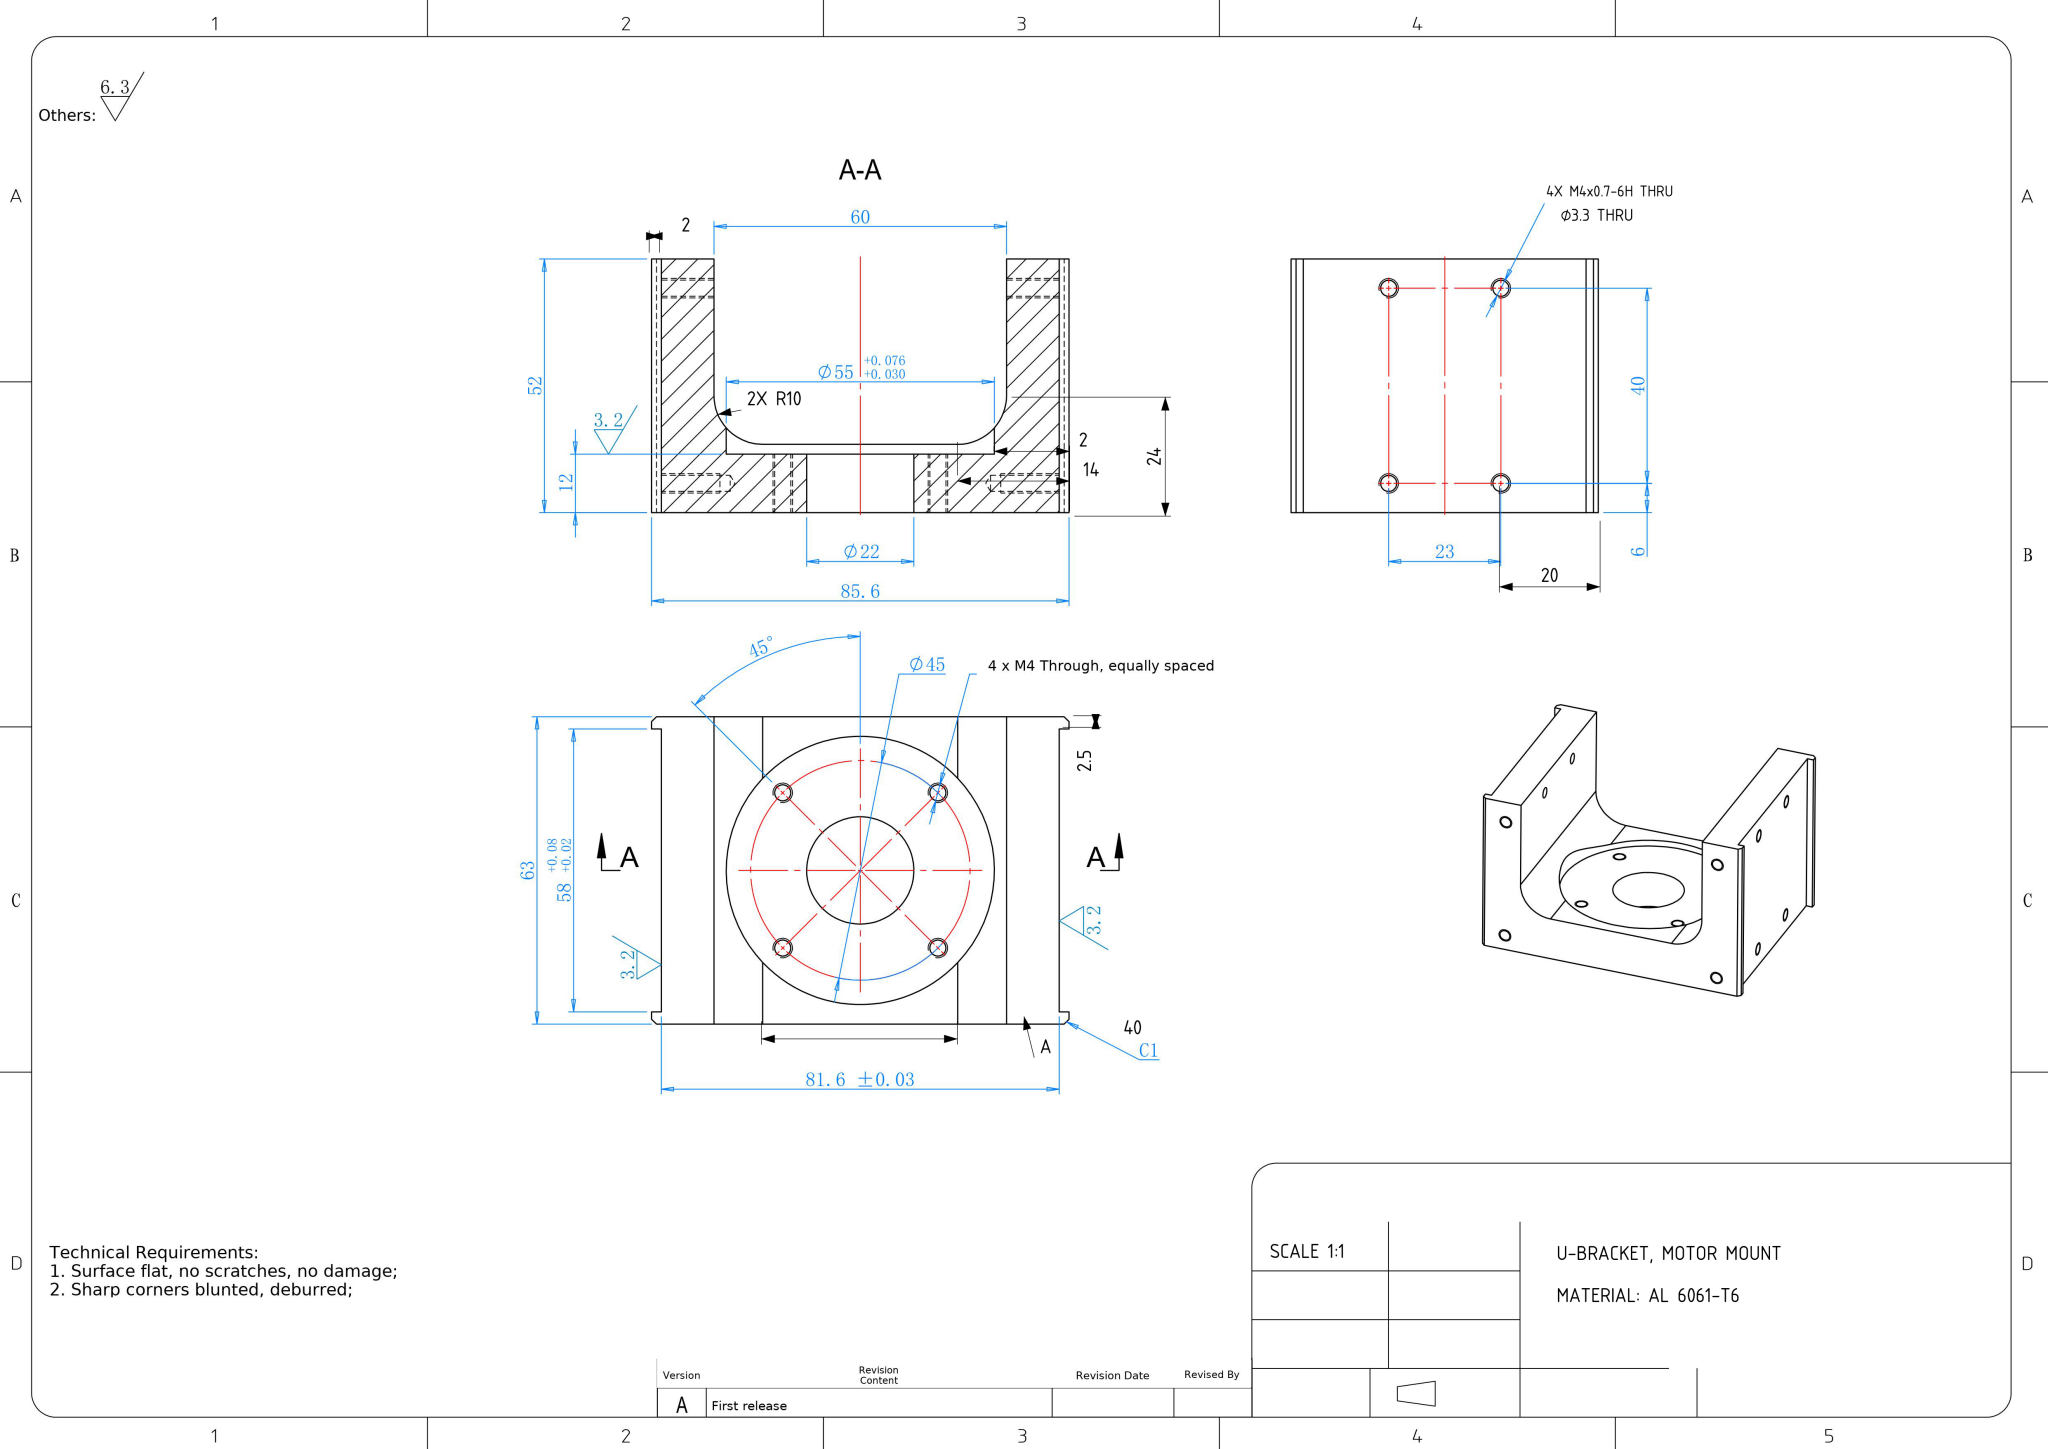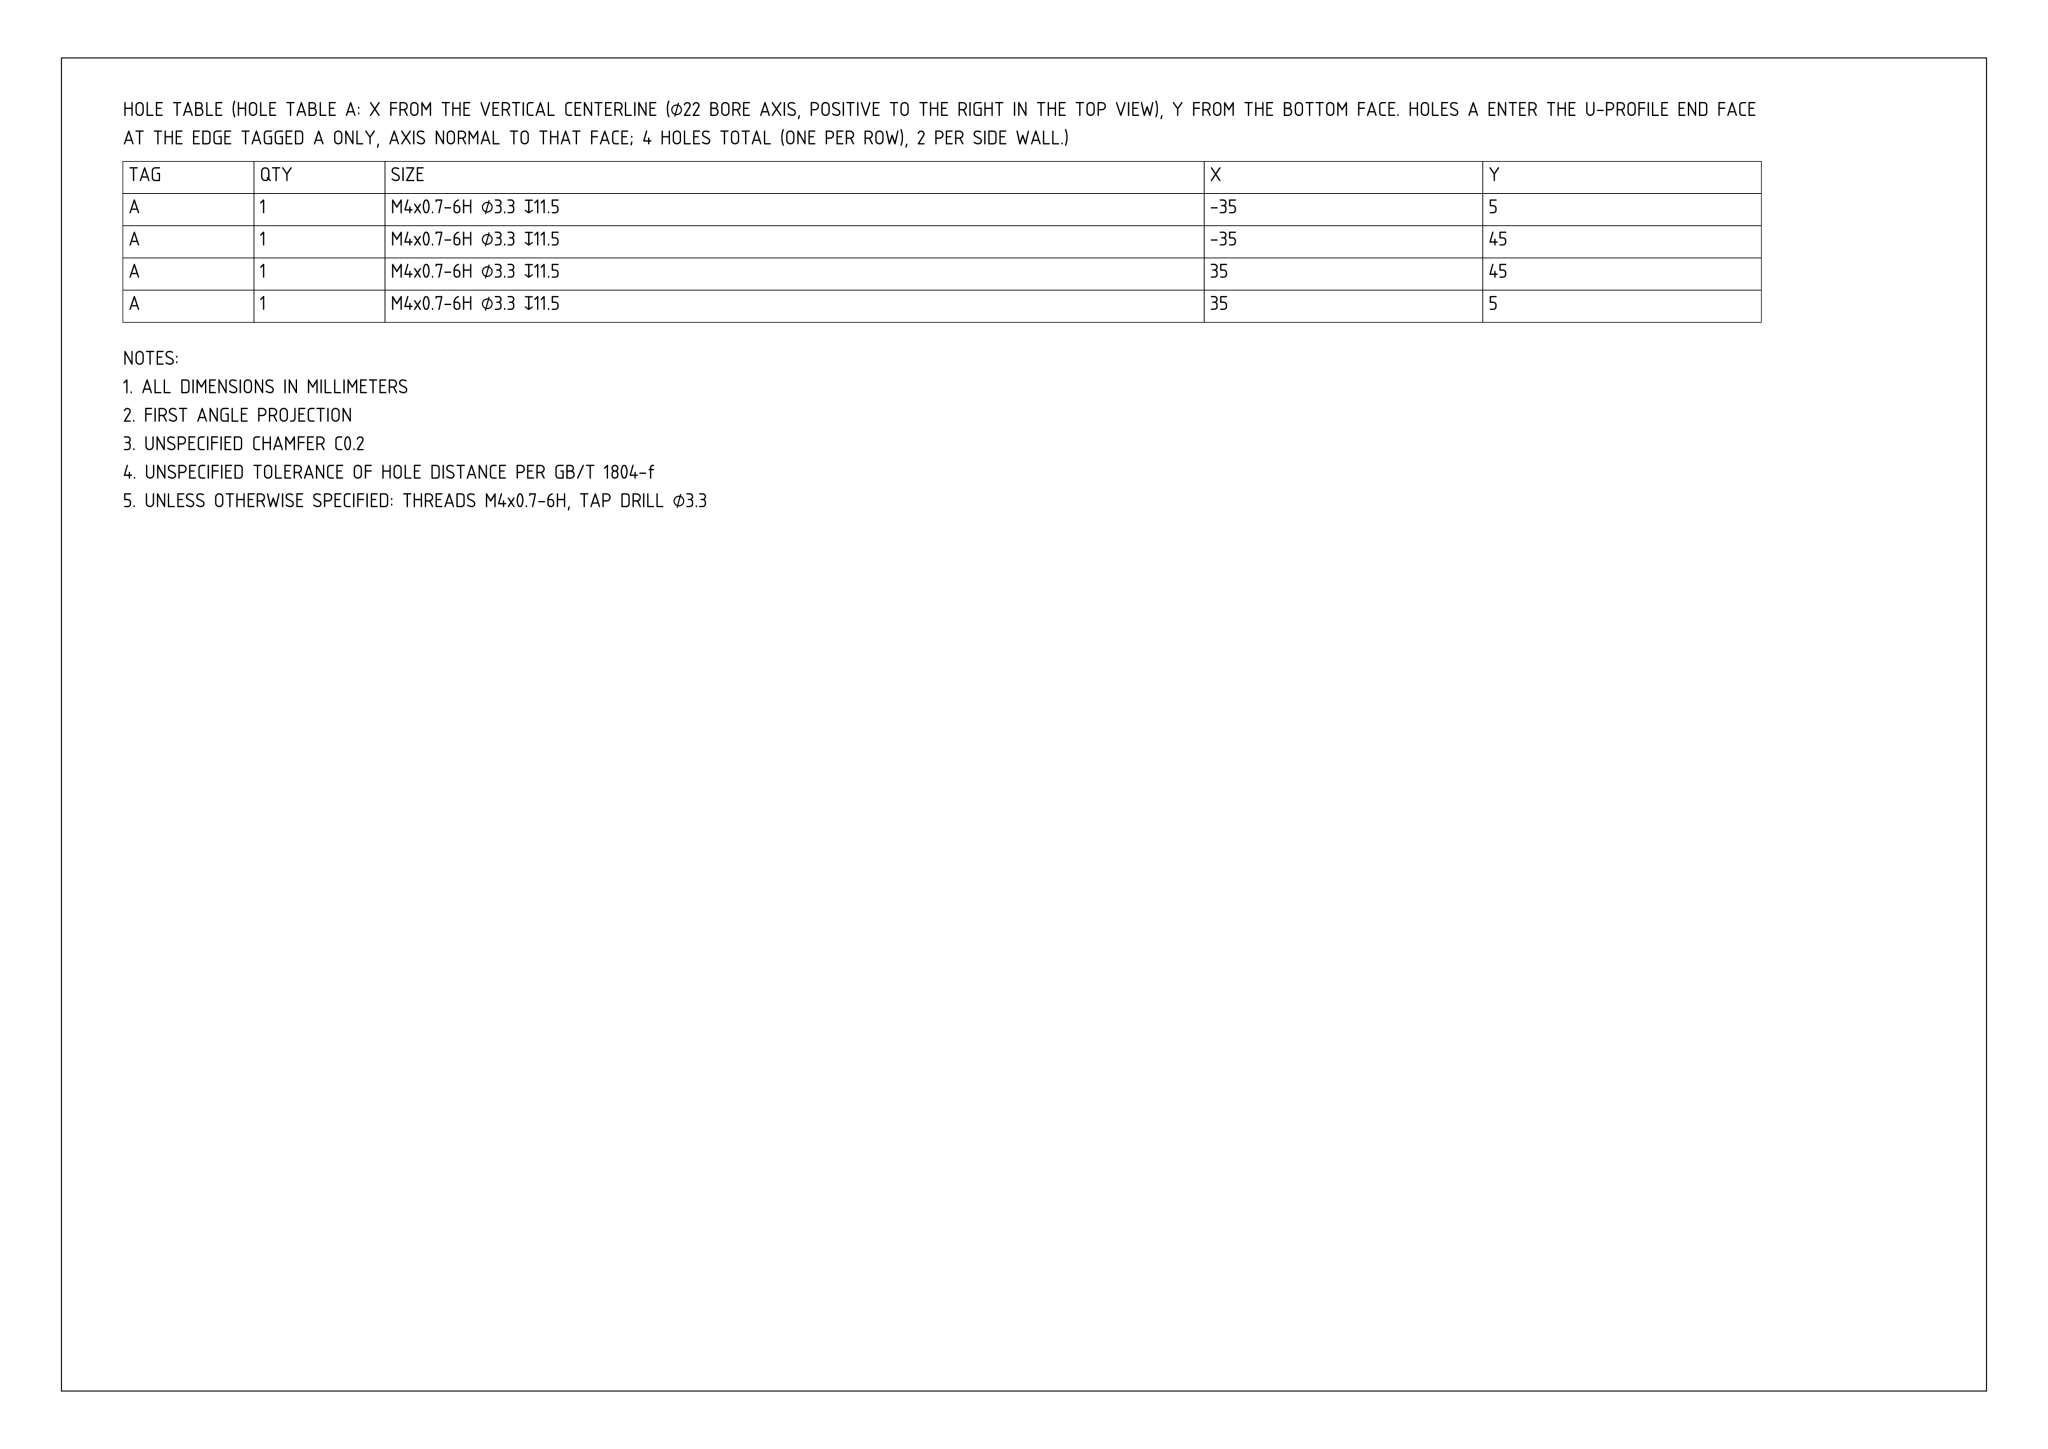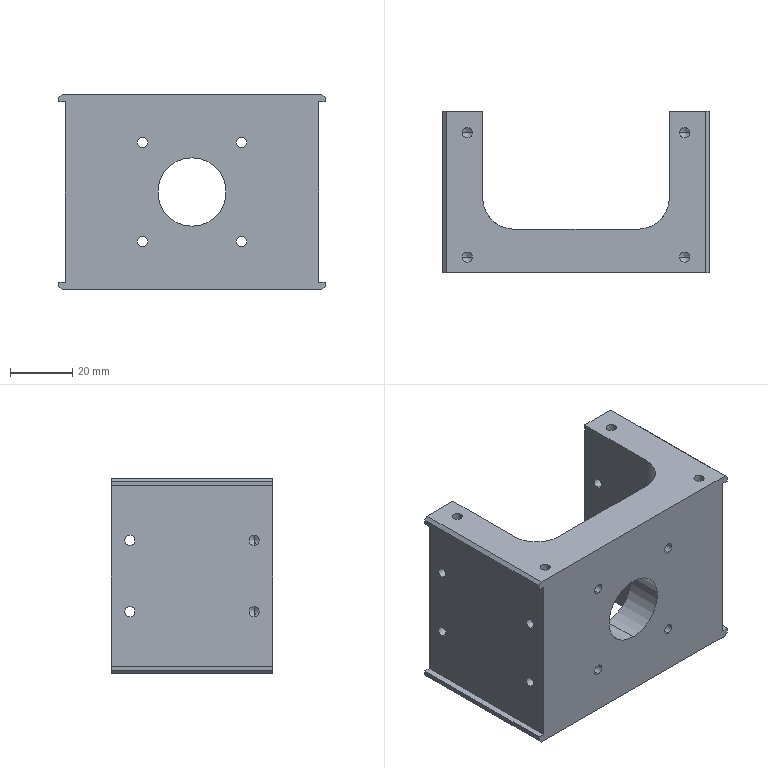Part | NX | mm | U-Notched Cylindrical Bearing Housing | 1 solid | 78 faces | box 85.6 x 52 x 63 mm | volume 116053 mm3 | cylinder 38 | plane 24 | cone 16 | commonest cylinder face diameters 3.3 x32 55 x2 22 x2 20 x2